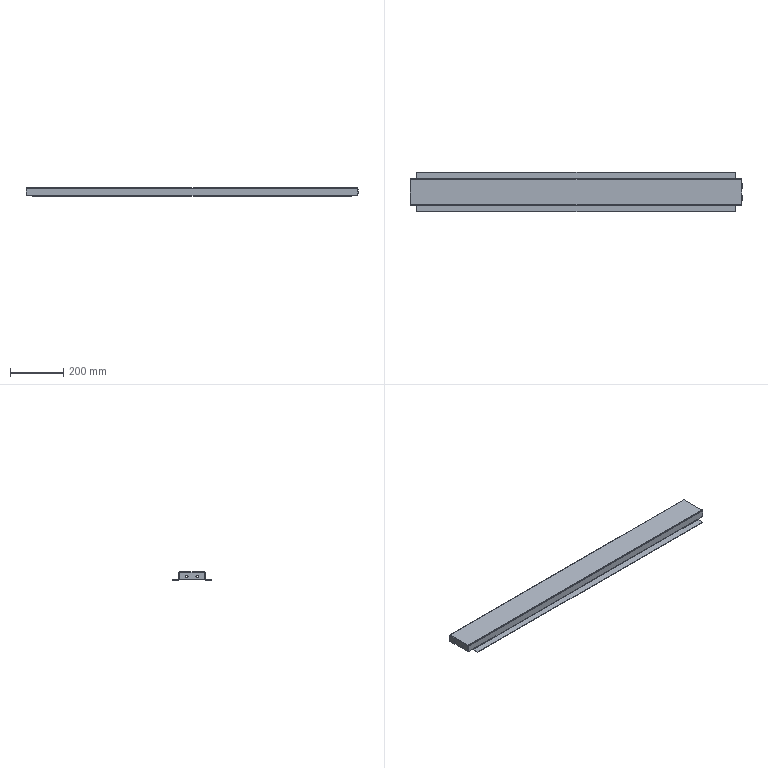Component | SolidWorks | 28FrontMiddleBeam-1 | 1 solid | 70 faces | volume 519595 mm3 | plane 50 | cylinder 20 | commonest cylinder face diameters 10 x8 6 x6 2 x6